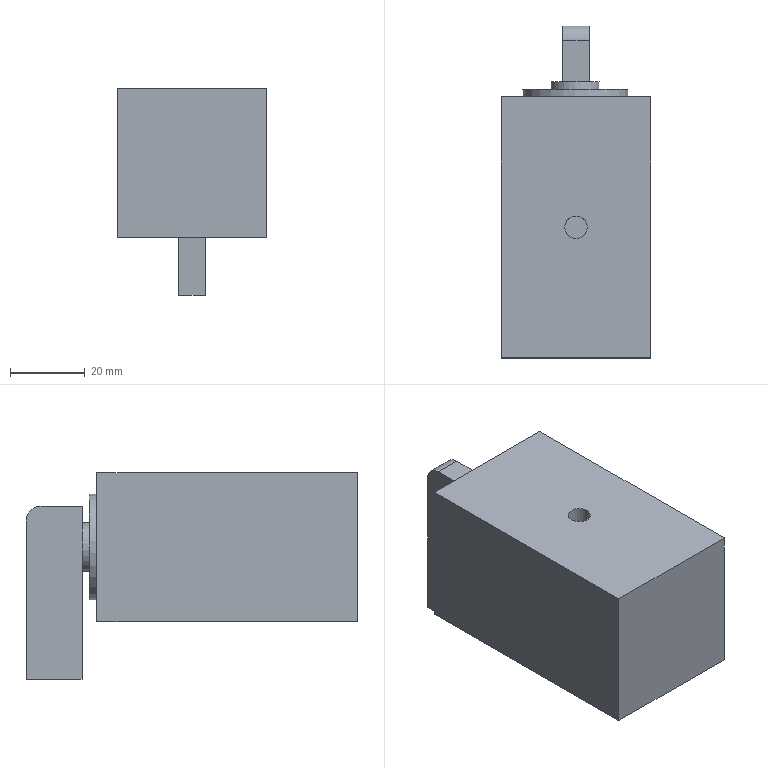Component | NX | MAG_BASE | 4 solids | 21 faces | volume 118101 mm3 | plane 17 | cylinder 4 | commonest cylinder face diameters 6 x1 8 x1 13.052 x1 28.3 x1